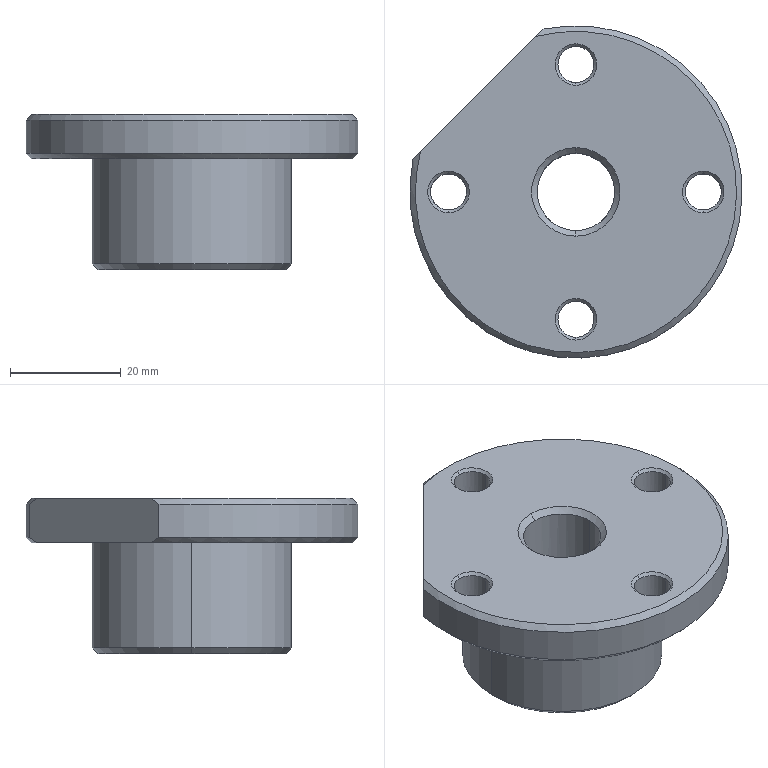CAM job | Mastercam | mm | 3 operations | part box 60 x 60 x 28
1. Contour (Ramp) | 9 - 8 平铣刀
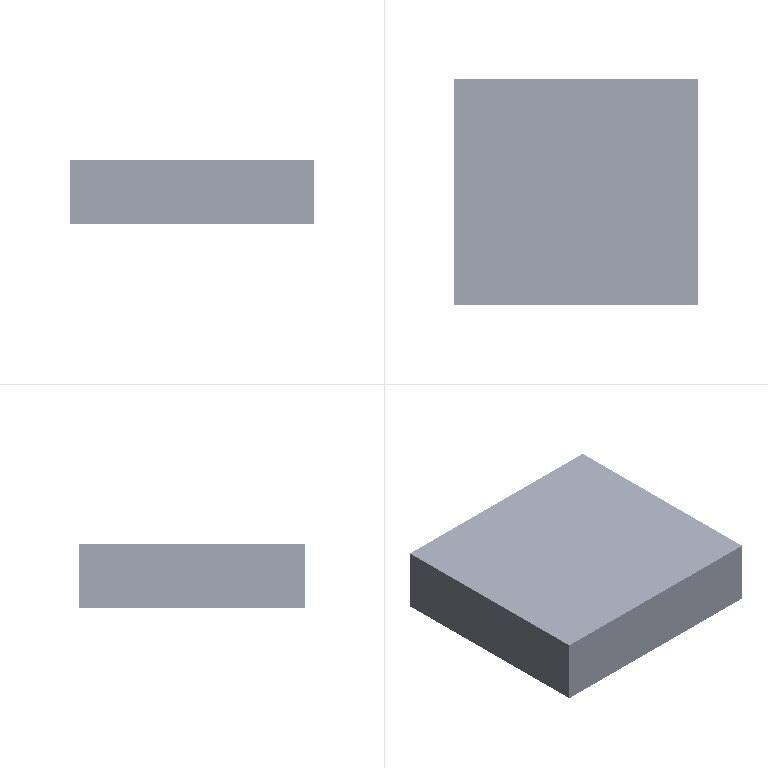2. Contour (2D) | 9 - 8 平铣刀
3. Drill/Counterbore | 7 - 4 倒角刀